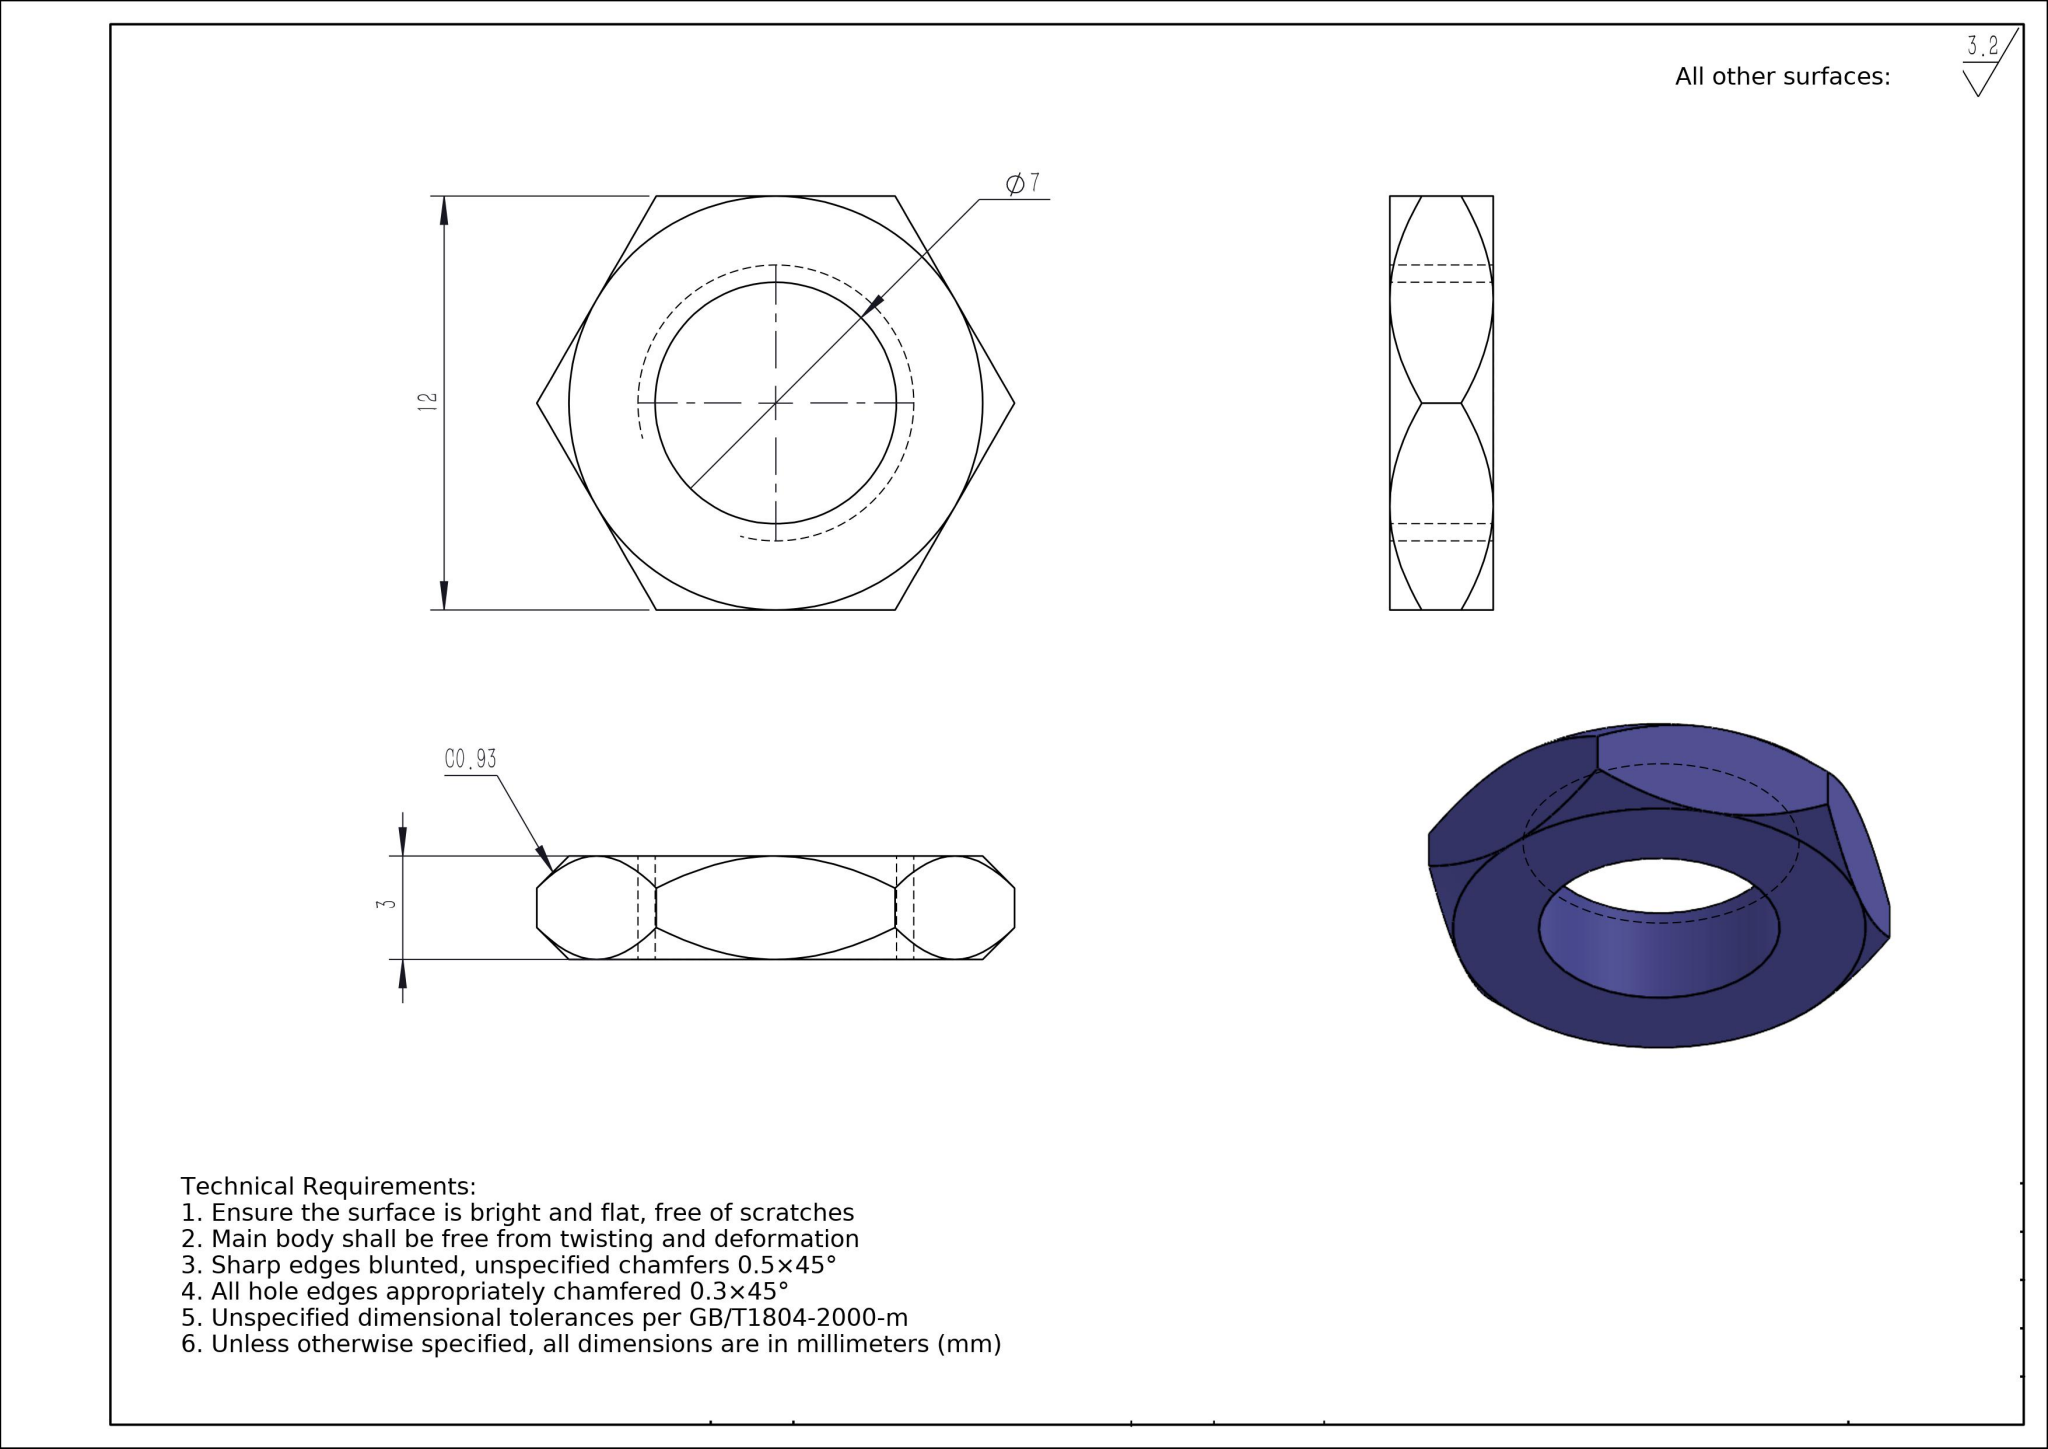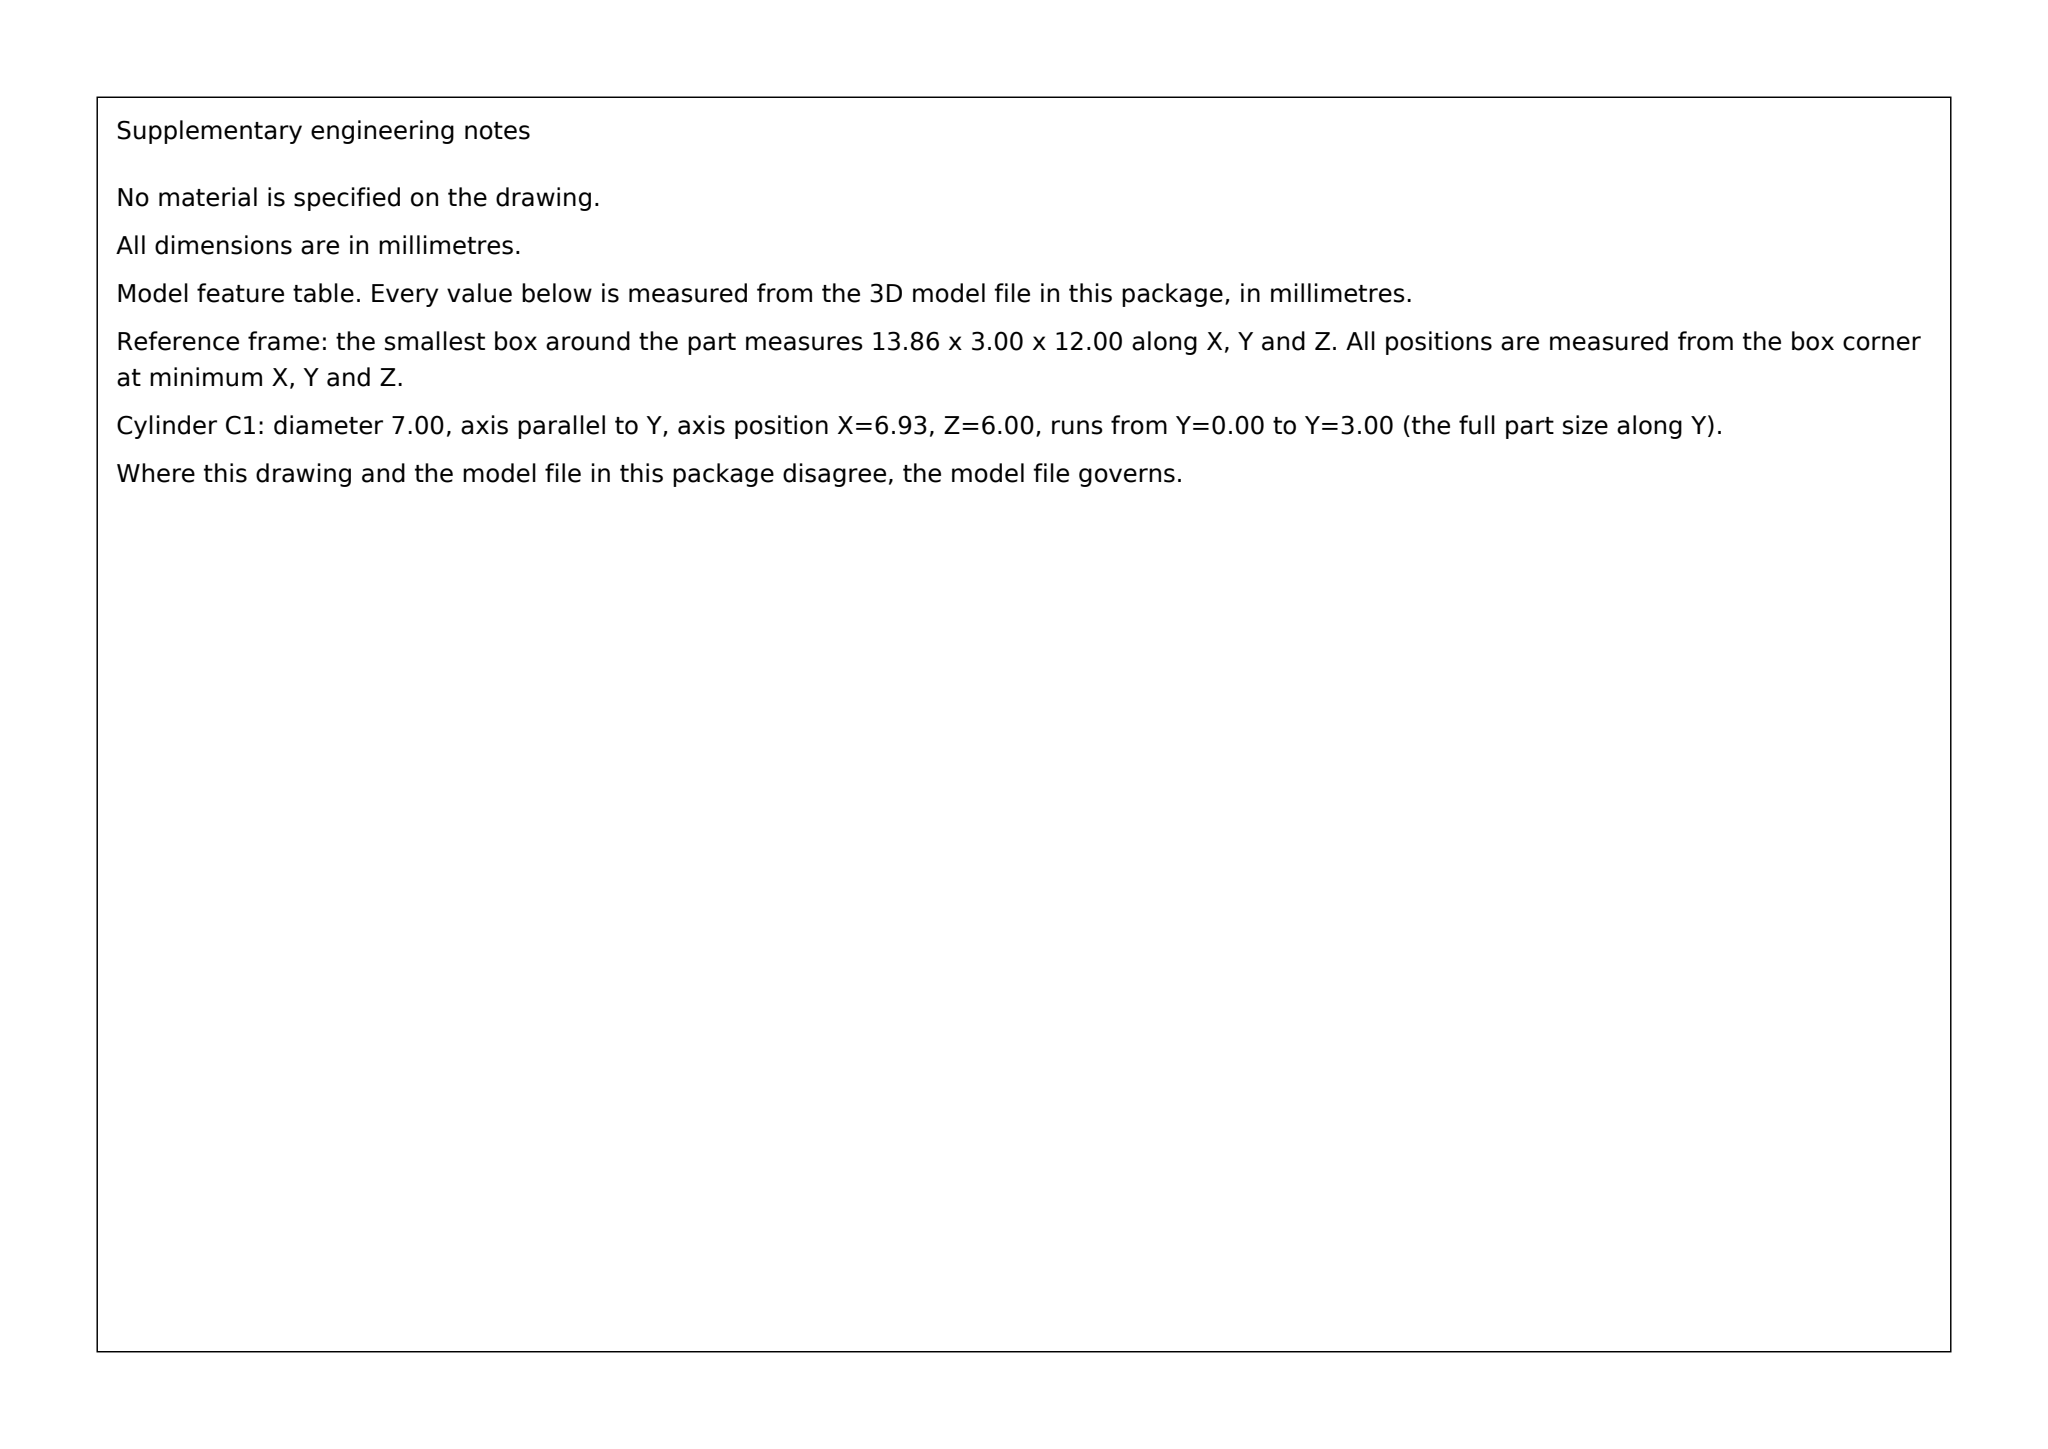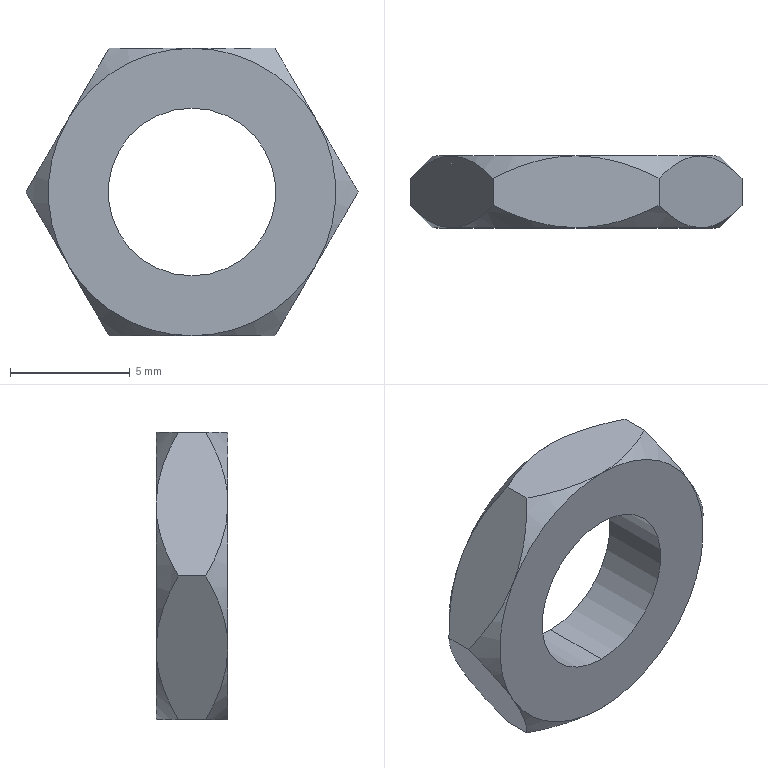Part | SolidWorks | mm | 1 solid | 22 faces | box 13.86 x 3 x 12 mm | volume 252 mm3 | cone 12 | plane 8 | cylinder 2 | commonest cylinder face diameters 7 x2
build123d program:
from build123d import *

# Parameters (mm, degrees)
BOSS_EXTRUDE2_DEPTH       = 3
M8X1_0_TAPPED_HOLE1_D     = 7
M8X1_0_TAPPED_HOLE1_DEPTH = 19
M8X1_0_TAPPED_HOLE1_TIP   = 2.103
SKETCH4_OUTSIDE_W         = 25.57
SKETCH4_OUTSIDE_H         = 23.714
SKETCH4_OUTSIDE_R         = 6
CUT_EXTRUDE1_DEPTH        = 3
CUT_EXTRUDE1_DRAFT        = -45
SKETCH5_OUTSIDE_W         = 25.57
SKETCH5_OUTSIDE_H         = 23.714
SKETCH5_OUTSIDE_R         = 6
CUT_EXTRUDE2_DEPTH        = 3
CUT_EXTRUDE2_DRAFT        = -45


with BuildPart() as part:
    # Sketch1 → Boss-Extrude2 (new body)
    with BuildSketch(Plane(origin=(0, 0, 0), x_dir=(1, 0, 0), z_dir=(0, 1, 0))):
        Polygon((6.928, 0), (3.464, 6), (-3.464, 6), (-6.928, 0), (-3.464, -6), (3.464, -6), align=None)
    extrude(amount=BOSS_EXTRUDE2_DEPTH)

    # M8x1.0 Tapped Hole1
    with Locations(Plane(origin=(0, 3, 0), x_dir=(1, 0, 0), z_dir=(0, 1, 0))):
        with Locations((0, 0)):
            Hole(M8X1_0_TAPPED_HOLE1_D / 2, depth=M8X1_0_TAPPED_HOLE1_DEPTH)
            with Locations((0, 0, -(M8X1_0_TAPPED_HOLE1_DEPTH + M8X1_0_TAPPED_HOLE1_TIP / 2))):  # 118° drill point
                Cone(0, M8X1_0_TAPPED_HOLE1_D / 2, M8X1_0_TAPPED_HOLE1_TIP, mode=Mode.SUBTRACT)


with BuildPart() as cut_extrude1_tool:
    # Sketch4 outside → Cut-Extrude1 (with draft: the straight prism first)
    with BuildSketch(Plane(origin=(0, 3, 0), x_dir=(1, 0, 0), z_dir=(0, 1, 0))):
        Rectangle(SKETCH4_OUTSIDE_W, SKETCH4_OUTSIDE_H)
        Circle(SKETCH4_OUTSIDE_R, mode=Mode.SUBTRACT)
    extrude(amount=-CUT_EXTRUDE1_DEPTH)
    # Cut-Extrude1: the draft: its side faces are tilted about the plane it starts from
    cut_extrude1_sides = [cut_extrude1_tool.faces().sort_by_distance(p)[0] for p in [
        (0, 1.5, 11.857),
        (12.785, 1.5, 0),
        (0, 1.5, -11.857),
        (-12.785, 1.5, 0),
        (-6, 1.5, 0),
    ]]
    draft(cut_extrude1_sides, Plane(origin=(0, 3, 0), x_dir=(1, 0, 0), z_dir=(0, 1, 0)), CUT_EXTRUDE1_DRAFT)


with BuildPart() as part_1:
    add(part.part)

    # Cut-Extrude1: cut by cut_extrude1_tool
    add(cut_extrude1_tool.part, mode=Mode.SUBTRACT)


with BuildPart() as cut_extrude2_tool:
    # Sketch5 outside → Cut-Extrude2 (with draft: the straight prism first)
    with BuildSketch(Plane.XZ):
        Rectangle(SKETCH5_OUTSIDE_W, SKETCH5_OUTSIDE_H)
        Circle(SKETCH5_OUTSIDE_R, mode=Mode.SUBTRACT)
    extrude(amount=-CUT_EXTRUDE2_DEPTH)
    # Cut-Extrude2: the draft: its side faces are tilted about the plane it starts from
    cut_extrude2_sides = [cut_extrude2_tool.faces().sort_by_distance(p)[0] for p in [
        (0, 1.5, -11.857),
        (12.785, 1.5, 0),
        (0, 1.5, 11.857),
        (-12.785, 1.5, 0),
        (-6, 1.5, 0),
    ]]
    draft(cut_extrude2_sides, Plane.XZ, CUT_EXTRUDE2_DRAFT)


with BuildPart() as part_2:
    add(part_1.part)

    # Cut-Extrude2: cut by cut_extrude2_tool
    add(cut_extrude2_tool.part, mode=Mode.SUBTRACT)


solid = part_2.part
STEP:
#1=CARTESIAN_POINT('',(0.,0.,-3.5));
#2=VERTEX_POINT('',#1);
#3=CARTESIAN_POINT('',(0.,0.,3.5));
#4=VERTEX_POINT('',#3);
#5=CARTESIAN_POINT('',(0.,0.,0.));
#6=DIRECTION('',(0.,1.,0.));
#7=DIRECTION('',(0.,0.,1.));
#8=AXIS2_PLACEMENT_3D('',#5,#6,#7);
#9=CIRCLE('',#8,3.5);
#10=EDGE_CURVE('',#2,#4,#9,.T.);
#11=ORIENTED_EDGE('',*,*,#10,.F.);
#12=CARTESIAN_POINT('',(0.,3.,-3.5));
#13=VERTEX_POINT('',#12);
#14=CARTESIAN_POINT('',(0.,3.,-3.5));
#15=DIRECTION('',(0.,1.,0.));
#16=VECTOR('',#15,1000.);
#17=LINE('',#14,#16);
#18=EDGE_CURVE('',#2,#13,#17,.T.);
#19=ORIENTED_EDGE('',*,*,#18,.T.);
#20=CARTESIAN_POINT('',(0.,3.,3.5));
#21=VERTEX_POINT('',#20);
#22=CARTESIAN_POINT('',(0.,3.,0.));
#23=DIRECTION('',(0.,1.,0.));
#24=DIRECTION('',(0.,0.,1.));
#25=AXIS2_PLACEMENT_3D('',#22,#23,#24);
#26=CIRCLE('',#25,3.5);
#27=EDGE_CURVE('',#13,#21,#26,.T.);
#28=ORIENTED_EDGE('',*,*,#27,.T.);
#29=CARTESIAN_POINT('',(0.,3.,3.5));
#30=DIRECTION('',(0.,1.,0.));
#31=VECTOR('',#30,1000.);
#32=LINE('',#29,#31);
#33=EDGE_CURVE('',#4,#21,#32,.T.);
#34=ORIENTED_EDGE('',*,*,#33,.F.);
#35=EDGE_LOOP('',(#11,#19,#28,#34));
#36=FACE_OUTER_BOUND('',#35,.T.);
#37=CARTESIAN_POINT('',(0.,3.,0.));
#38=DIRECTION('',(0.,1.,0.));
#39=DIRECTION('',(0.,0.,1.));
#40=AXIS2_PLACEMENT_3D('',#37,#38,#39);
#41=CYLINDRICAL_SURFACE('',#40,3.5);
#42=ADVANCED_FACE('',(#36),#41,.F.);
#43=CARTESIAN_POINT('',(6.928,0.9282,0.));
#44=VERTEX_POINT('',#43);
#45=CARTESIAN_POINT('',(5.196,0.,3.));
#46=VERTEX_POINT('',#45);
#47=CARTESIAN_POINT('',(6.928,0.9282,0.));
#48=CARTESIAN_POINT('',(6.657,0.6566,0.4704));
#49=CARTESIAN_POINT('',(6.379,0.4258,0.9515));
#50=CARTESIAN_POINT('',(5.947,0.179,1.699));
#51=CARTESIAN_POINT('',(5.801,0.1135,1.953));
#52=CARTESIAN_POINT('',(5.502,0.02381,2.471));
#53=CARTESIAN_POINT('',(5.348,0.,2.737));
#54=CARTESIAN_POINT('',(5.196,0.,3.));
#55=B_SPLINE_CURVE_WITH_KNOTS('',3,(#47,#48,#49,#50,#51,#52,#53,#54),.UNSPECIFIED.,.F.,.F.,(4,2,2,4),(0.00000025,0.001796,0.002693,0.003591),.UNSPECIFIED.);
#56=EDGE_CURVE('',#44,#46,#55,.T.);
#57=ORIENTED_EDGE('',*,*,#56,.F.);
#58=CARTESIAN_POINT('',(6.928,2.072,0.));
#59=VERTEX_POINT('',#58);
#60=CARTESIAN_POINT('',(6.928,3.,0.));
#61=DIRECTION('',(0.,-1.,0.));
#62=VECTOR('',#61,1000.);
#63=LINE('',#60,#62);
#64=EDGE_CURVE('',#59,#44,#63,.T.);
#65=ORIENTED_EDGE('',*,*,#64,.F.);
#66=CARTESIAN_POINT('',(5.196,3.,3.));
#67=VERTEX_POINT('',#66);
#68=CARTESIAN_POINT('',(5.196,3.,3.));
#69=CARTESIAN_POINT('',(5.497,3.,2.478));
#70=CARTESIAN_POINT('',(5.794,2.908,1.965));
#71=CARTESIAN_POINT('',(6.378,2.576,0.9536));
#72=CARTESIAN_POINT('',(6.657,2.343,0.4699));
#73=CARTESIAN_POINT('',(6.928,2.072,0.));
#74=B_SPLINE_CURVE_WITH_KNOTS('',3,(#68,#69,#70,#71,#72,#73),.UNSPECIFIED.,.F.,.F.,(4,2,4),(0.003591,0.005374,0.007157),.UNSPECIFIED.);
#75=EDGE_CURVE('',#67,#59,#74,.T.);
#76=ORIENTED_EDGE('',*,*,#75,.F.);
#77=CARTESIAN_POINT('',(3.464,2.072,6.));
#78=VERTEX_POINT('',#77);
#79=CARTESIAN_POINT('',(3.464,2.072,6.));
#80=CARTESIAN_POINT('',(3.736,2.343,5.53));
#81=CARTESIAN_POINT('',(4.013,2.574,5.048));
#82=CARTESIAN_POINT('',(4.445,2.821,4.301));
#83=CARTESIAN_POINT('',(4.591,2.886,4.047));
#84=CARTESIAN_POINT('',(4.89,2.976,3.529));
#85=CARTESIAN_POINT('',(5.044,3.,3.263));
#86=CARTESIAN_POINT('',(5.196,3.,3.));
#87=B_SPLINE_CURVE_WITH_KNOTS('',3,(#79,#80,#81,#82,#83,#84,#85,#86),.UNSPECIFIED.,.F.,.F.,(4,2,2,4),(0.00000025,0.001796,0.002693,0.003591),.UNSPECIFIED.);
#88=EDGE_CURVE('',#78,#67,#87,.T.);
#89=ORIENTED_EDGE('',*,*,#88,.F.);
#90=CARTESIAN_POINT('',(3.464,0.9282,6.));
#91=VERTEX_POINT('',#90);
#92=CARTESIAN_POINT('',(3.464,3.,6.));
#93=DIRECTION('',(0.,-1.,0.));
#94=VECTOR('',#93,1000.);
#95=LINE('',#92,#94);
#96=EDGE_CURVE('',#78,#91,#95,.T.);
#97=ORIENTED_EDGE('',*,*,#96,.T.);
#98=CARTESIAN_POINT('',(5.196,0.,3.));
#99=CARTESIAN_POINT('',(4.895,0.,3.522));
#100=CARTESIAN_POINT('',(4.599,0.09213,4.035));
#101=CARTESIAN_POINT('',(4.015,0.4242,5.046));
#102=CARTESIAN_POINT('',(3.735,0.6569,5.53));
#103=CARTESIAN_POINT('',(3.464,0.9282,6.));
#104=B_SPLINE_CURVE_WITH_KNOTS('',3,(#98,#99,#100,#101,#102,#103),.UNSPECIFIED.,.F.,.F.,(4,2,4),(0.003591,0.005374,0.007157),.UNSPECIFIED.);
#105=EDGE_CURVE('',#46,#91,#104,.T.);
#106=ORIENTED_EDGE('',*,*,#105,.F.);
#107=EDGE_LOOP('',(#57,#65,#76,#89,#97,#106));
#108=FACE_OUTER_BOUND('',#107,.T.);
#109=CARTESIAN_POINT('',(3.464,3.,6.));
#110=DIRECTION('',(-0.866,0.,-0.5));
#111=DIRECTION('',(-0.5,0.,0.866));
#112=AXIS2_PLACEMENT_3D('',#109,#110,#111);
#113=PLANE('',#112);
#114=ADVANCED_FACE('',(#108),#113,.F.);
#115=CARTESIAN_POINT('',(3.464,0.9282,-6.));
#116=VERTEX_POINT('',#115);
#117=CARTESIAN_POINT('',(5.196,0.,-3.));
#118=VERTEX_POINT('',#117);
#119=CARTESIAN_POINT('',(3.464,0.9282,-6.));
#120=CARTESIAN_POINT('',(3.736,0.6566,-5.53));
#121=CARTESIAN_POINT('',(4.013,0.4258,-5.048));
#122=CARTESIAN_POINT('',(4.445,0.179,-4.301));
#123=CARTESIAN_POINT('',(4.591,0.1135,-4.047));
#124=CARTESIAN_POINT('',(4.89,0.02381,-3.529));
#125=CARTESIAN_POINT('',(5.044,-0.,-3.263));
#126=CARTESIAN_POINT('',(5.196,0.,-3.));
#127=B_SPLINE_CURVE_WITH_KNOTS('',3,(#119,#120,#121,#122,#123,#124,#125,#126),.UNSPECIFIED.,.F.,.F.,(4,2,2,4),(0.00000025,0.001796,0.002693,0.003591),.UNSPECIFIED.);
#128=EDGE_CURVE('',#116,#118,#127,.T.);
#129=ORIENTED_EDGE('',*,*,#128,.F.);
#130=CARTESIAN_POINT('',(3.464,2.072,-6.));
#131=VERTEX_POINT('',#130);
#132=CARTESIAN_POINT('',(3.464,3.,-6.));
#133=DIRECTION('',(0.,-1.,0.));
#134=VECTOR('',#133,1000.);
#135=LINE('',#132,#134);
#136=EDGE_CURVE('',#131,#116,#135,.T.);
#137=ORIENTED_EDGE('',*,*,#136,.F.);
#138=CARTESIAN_POINT('',(5.196,3.,-3.));
#139=VERTEX_POINT('',#138);
#140=CARTESIAN_POINT('',(5.196,3.,-3.));
#141=CARTESIAN_POINT('',(4.895,3.,-3.522));
#142=CARTESIAN_POINT('',(4.599,2.908,-4.035));
#143=CARTESIAN_POINT('',(4.015,2.576,-5.046));
#144=CARTESIAN_POINT('',(3.735,2.343,-5.53));
#145=CARTESIAN_POINT('',(3.464,2.072,-6.));
#146=B_SPLINE_CURVE_WITH_KNOTS('',3,(#140,#141,#142,#143,#144,#145),.UNSPECIFIED.,.F.,.F.,(4,2,4),(0.003591,0.005374,0.007157),.UNSPECIFIED.);
#147=EDGE_CURVE('',#139,#131,#146,.T.);
#148=ORIENTED_EDGE('',*,*,#147,.F.);
#149=CARTESIAN_POINT('',(6.928,2.072,0.));
#150=CARTESIAN_POINT('',(6.657,2.343,-0.4704));
#151=CARTESIAN_POINT('',(6.379,2.574,-0.9515));
#152=CARTESIAN_POINT('',(5.947,2.821,-1.699));
#153=CARTESIAN_POINT('',(5.801,2.886,-1.953));
#154=CARTESIAN_POINT('',(5.502,2.976,-2.471));
#155=CARTESIAN_POINT('',(5.348,3.,-2.737));
#156=CARTESIAN_POINT('',(5.196,3.,-3.));
#157=B_SPLINE_CURVE_WITH_KNOTS('',3,(#149,#150,#151,#152,#153,#154,#155,#156),.UNSPECIFIED.,.F.,.F.,(4,2,2,4),(0.00000025,0.001796,0.002693,0.003591),.UNSPECIFIED.);
#158=EDGE_CURVE('',#59,#139,#157,.T.);
#159=ORIENTED_EDGE('',*,*,#158,.F.);
#160=ORIENTED_EDGE('',*,*,#64,.T.);
#161=CARTESIAN_POINT('',(5.196,0.,-3.));
#162=CARTESIAN_POINT('',(5.497,-0.,-2.478));
#163=CARTESIAN_POINT('',(5.794,0.09213,-1.965));
#164=CARTESIAN_POINT('',(6.378,0.4242,-0.9536));
#165=CARTESIAN_POINT('',(6.657,0.6569,-0.4699));
#166=CARTESIAN_POINT('',(6.928,0.9282,0.));
#167=B_SPLINE_CURVE_WITH_KNOTS('',3,(#161,#162,#163,#164,#165,#166),.UNSPECIFIED.,.F.,.F.,(4,2,4),(0.003591,0.005374,0.007157),.UNSPECIFIED.);
#168=EDGE_CURVE('',#118,#44,#167,.T.);
#169=ORIENTED_EDGE('',*,*,#168,.F.);
#170=EDGE_LOOP('',(#129,#137,#148,#159,#160,#169));
#171=FACE_OUTER_BOUND('',#170,.T.);
#172=CARTESIAN_POINT('',(6.928,3.,0.));
#173=DIRECTION('',(-0.866,0.,0.5));
#174=DIRECTION('',(0.5,0.,0.866));
#175=AXIS2_PLACEMENT_3D('',#172,#173,#174);
#176=PLANE('',#175);
#177=ADVANCED_FACE('',(#171),#176,.F.);
#178=CARTESIAN_POINT('',(-3.464,0.9282,-6.));
#179=VERTEX_POINT('',#178);
#180=CARTESIAN_POINT('',(0.,0.,-6.));
#181=VERTEX_POINT('',#180);
#182=CARTESIAN_POINT('',(-3.464,0.9282,-6.));
#183=CARTESIAN_POINT('',(-2.927,0.6597,-6.));
#184=CARTESIAN_POINT('',(-2.362,0.4243,-6.));
#185=CARTESIAN_POINT('',(-1.496,0.1774,-6.));
#186=CARTESIAN_POINT('',(-1.203,0.1123,-6.));
#187=CARTESIAN_POINT('',(-0.6083,0.02359,-6.));
#188=CARTESIAN_POINT('',(-0.3039,-0.,-6.));
#189=CARTESIAN_POINT('',(0.,0.,-6.));
#190=B_SPLINE_CURVE_WITH_KNOTS('',3,(#182,#183,#184,#185,#186,#187,#188,#189),.UNSPECIFIED.,.F.,.F.,(4,2,2,4),(0.006042,0.00783,0.008725,0.009619),.UNSPECIFIED.);
#191=EDGE_CURVE('',#179,#181,#190,.T.);
#192=ORIENTED_EDGE('',*,*,#191,.F.);
#193=CARTESIAN_POINT('',(-3.464,2.072,-6.));
#194=VERTEX_POINT('',#193);
#195=CARTESIAN_POINT('',(-3.464,3.,-6.));
#196=DIRECTION('',(0.,-1.,0.));
#197=VECTOR('',#196,1000.);
#198=LINE('',#195,#197);
#199=EDGE_CURVE('',#194,#179,#198,.T.);
#200=ORIENTED_EDGE('',*,*,#199,.F.);
#201=CARTESIAN_POINT('',(0.,3.,-6.));
#202=VERTEX_POINT('',#201);
#203=CARTESIAN_POINT('',(0.,3.,-6.));
#204=CARTESIAN_POINT('',(-0.3039,3.,-6.));
#205=CARTESIAN_POINT('',(-0.6083,2.976,-6.));
#206=CARTESIAN_POINT('',(-1.203,2.888,-6.));
#207=CARTESIAN_POINT('',(-1.496,2.823,-6.));
#208=CARTESIAN_POINT('',(-2.362,2.576,-6.));
#209=CARTESIAN_POINT('',(-2.927,2.34,-6.));
#210=CARTESIAN_POINT('',(-3.464,2.072,-6.));
#211=B_SPLINE_CURVE_WITH_KNOTS('',3,(#203,#204,#205,#206,#207,#208,#209,#210),.UNSPECIFIED.,.F.,.F.,(4,2,2,4),(0.007239,0.008136,0.009033,0.01083),.UNSPECIFIED.);
#212=EDGE_CURVE('',#202,#194,#211,.T.);
#213=ORIENTED_EDGE('',*,*,#212,.F.);
#214=CARTESIAN_POINT('',(3.464,2.072,-6.));
#215=CARTESIAN_POINT('',(3.196,2.206,-6.));
#216=CARTESIAN_POINT('',(2.923,2.331,-6.));
#217=CARTESIAN_POINT('',(2.362,2.557,-6.));
#218=CARTESIAN_POINT('',(2.073,2.658,-6.));
#219=CARTESIAN_POINT('',(1.202,2.906,-6.));
#220=CARTESIAN_POINT('',(0.6086,3.,-6.));
#221=CARTESIAN_POINT('',(0.,3.,-6.));
#222=B_SPLINE_CURVE_WITH_KNOTS('',3,(#214,#215,#216,#217,#218,#219,#220,#221),.UNSPECIFIED.,.F.,.F.,(4,2,2,4),(0.003647,0.004545,0.005443,0.007239),.UNSPECIFIED.);
#223=EDGE_CURVE('',#131,#202,#222,.T.);
#224=ORIENTED_EDGE('',*,*,#223,.F.);
#225=ORIENTED_EDGE('',*,*,#136,.T.);
#226=CARTESIAN_POINT('',(0.,0.,-6.));
#227=CARTESIAN_POINT('',(0.6086,-0.,-6.));
#228=CARTESIAN_POINT('',(1.202,0.09373,-6.));
#229=CARTESIAN_POINT('',(2.073,0.3419,-6.));
#230=CARTESIAN_POINT('',(2.362,0.443,-6.));
#231=CARTESIAN_POINT('',(2.923,0.669,-6.));
#232=CARTESIAN_POINT('',(3.196,0.7941,-6.));
#233=CARTESIAN_POINT('',(3.464,0.9282,-6.));
#234=B_SPLINE_CURVE_WITH_KNOTS('',3,(#226,#227,#228,#229,#230,#231,#232,#233),.UNSPECIFIED.,.F.,.F.,(4,2,2,4),(0.009619,0.01141,0.0123,0.0132),.UNSPECIFIED.);
#235=EDGE_CURVE('',#181,#116,#234,.T.);
#236=ORIENTED_EDGE('',*,*,#235,.F.);
#237=EDGE_LOOP('',(#192,#200,#213,#224,#225,#236));
#238=FACE_OUTER_BOUND('',#237,.T.);
#239=CARTESIAN_POINT('',(3.464,3.,-6.));
#240=DIRECTION('',(0.,0.,1.));
#241=DIRECTION('',(1.,0.,0.));
#242=AXIS2_PLACEMENT_3D('',#239,#240,#241);
#243=PLANE('',#242);
#244=ADVANCED_FACE('',(#238),#243,.F.);
#245=CARTESIAN_POINT('',(-6.928,0.9282,0.));
#246=VERTEX_POINT('',#245);
#247=CARTESIAN_POINT('',(-5.196,0.,-3.));
#248=VERTEX_POINT('',#247);
#249=CARTESIAN_POINT('',(-6.928,0.9282,0.));
#250=CARTESIAN_POINT('',(-6.657,0.6566,-0.4704));
#251=CARTESIAN_POINT('',(-6.379,0.4258,-0.9515));
#252=CARTESIAN_POINT('',(-5.947,0.179,-1.699));
#253=CARTESIAN_POINT('',(-5.801,0.1135,-1.953));
#254=CARTESIAN_POINT('',(-5.502,0.02381,-2.471));
#255=CARTESIAN_POINT('',(-5.348,0.,-2.737));
#256=CARTESIAN_POINT('',(-5.196,0.,-3.));
#257=B_SPLINE_CURVE_WITH_KNOTS('',3,(#249,#250,#251,#252,#253,#254,#255,#256),.UNSPECIFIED.,.F.,.F.,(4,2,2,4),(0.00000025,0.001796,0.002693,0.003591),.UNSPECIFIED.);
#258=EDGE_CURVE('',#246,#248,#257,.T.);
#259=ORIENTED_EDGE('',*,*,#258,.F.);
#260=CARTESIAN_POINT('',(-6.928,2.072,0.));
#261=VERTEX_POINT('',#260);
#262=CARTESIAN_POINT('',(-6.928,3.,-0.));
#263=DIRECTION('',(0.,-1.,0.));
#264=VECTOR('',#263,1000.);
#265=LINE('',#262,#264);
#266=EDGE_CURVE('',#261,#246,#265,.T.);
#267=ORIENTED_EDGE('',*,*,#266,.F.);
#268=CARTESIAN_POINT('',(-5.196,3.,-3.));
#269=VERTEX_POINT('',#268);
#270=CARTESIAN_POINT('',(-5.196,3.,-3.));
#271=CARTESIAN_POINT('',(-5.497,3.,-2.478));
#272=CARTESIAN_POINT('',(-5.794,2.908,-1.965));
#273=CARTESIAN_POINT('',(-6.378,2.576,-0.9536));
#274=CARTESIAN_POINT('',(-6.657,2.343,-0.4699));
#275=CARTESIAN_POINT('',(-6.928,2.072,0.));
#276=B_SPLINE_CURVE_WITH_KNOTS('',3,(#270,#271,#272,#273,#274,#275),.UNSPECIFIED.,.F.,.F.,(4,2,4),(0.003591,0.005374,0.007157),.UNSPECIFIED.);
#277=EDGE_CURVE('',#269,#261,#276,.T.);
#278=ORIENTED_EDGE('',*,*,#277,.F.);
#279=CARTESIAN_POINT('',(-3.464,2.072,-6.));
#280=CARTESIAN_POINT('',(-3.736,2.343,-5.53));
#281=CARTESIAN_POINT('',(-4.013,2.574,-5.048));
#282=CARTESIAN_POINT('',(-4.445,2.821,-4.301));
#283=CARTESIAN_POINT('',(-4.591,2.886,-4.047));
#284=CARTESIAN_POINT('',(-4.89,2.976,-3.529));
#285=CARTESIAN_POINT('',(-5.044,3.,-3.263));
#286=CARTESIAN_POINT('',(-5.196,3.,-3.));
#287=B_SPLINE_CURVE_WITH_KNOTS('',3,(#279,#280,#281,#282,#283,#284,#285,#286),.UNSPECIFIED.,.F.,.F.,(4,2,2,4),(0.00000025,0.001796,0.002693,0.003591),.UNSPECIFIED.);
#288=EDGE_CURVE('',#194,#269,#287,.T.);
#289=ORIENTED_EDGE('',*,*,#288,.F.);
#290=ORIENTED_EDGE('',*,*,#199,.T.);
#291=CARTESIAN_POINT('',(-5.196,0.,-3.));
#292=CARTESIAN_POINT('',(-4.895,0.,-3.522));
#293=CARTESIAN_POINT('',(-4.599,0.09213,-4.035));
#294=CARTESIAN_POINT('',(-4.015,0.4242,-5.046));
#295=CARTESIAN_POINT('',(-3.735,0.6569,-5.53));
#296=CARTESIAN_POINT('',(-3.464,0.9282,-6.));
#297=B_SPLINE_CURVE_WITH_KNOTS('',3,(#291,#292,#293,#294,#295,#296),.UNSPECIFIED.,.F.,.F.,(4,2,4),(0.003591,0.005374,0.007157),.UNSPECIFIED.);
#298=EDGE_CURVE('',#248,#179,#297,.T.);
#299=ORIENTED_EDGE('',*,*,#298,.F.);
#300=EDGE_LOOP('',(#259,#267,#278,#289,#290,#299));
#301=FACE_OUTER_BOUND('',#300,.T.);
#302=CARTESIAN_POINT('',(-3.464,3.,-6.));
#303=DIRECTION('',(0.866,0.,0.5));
#304=DIRECTION('',(0.5,0.,-0.866));
#305=AXIS2_PLACEMENT_3D('',#302,#303,#304);
#306=PLANE('',#305);
#307=ADVANCED_FACE('',(#301),#306,.F.);
#308=CARTESIAN_POINT('',(-3.464,0.9282,6.));
#309=VERTEX_POINT('',#308);
#310=CARTESIAN_POINT('',(-5.196,0.,3.));
#311=VERTEX_POINT('',#310);
#312=CARTESIAN_POINT('',(-3.464,0.9282,6.));
#313=CARTESIAN_POINT('',(-3.736,0.6566,5.53));
#314=CARTESIAN_POINT('',(-4.013,0.4258,5.048));
#315=CARTESIAN_POINT('',(-4.445,0.179,4.301));
#316=CARTESIAN_POINT('',(-4.591,0.1135,4.047));
#317=CARTESIAN_POINT('',(-4.89,0.02381,3.529));
#318=CARTESIAN_POINT('',(-5.044,0.,3.263));
#319=CARTESIAN_POINT('',(-5.196,0.,3.));
#320=B_SPLINE_CURVE_WITH_KNOTS('',3,(#312,#313,#314,#315,#316,#317,#318,#319),.UNSPECIFIED.,.F.,.F.,(4,2,2,4),(0.00000025,0.001796,0.002693,0.003591),.UNSPECIFIED.);
#321=EDGE_CURVE('',#309,#311,#320,.T.);
#322=ORIENTED_EDGE('',*,*,#321,.F.);
#323=CARTESIAN_POINT('',(-3.464,2.072,6.));
#324=VERTEX_POINT('',#323);
#325=CARTESIAN_POINT('',(-3.464,3.,6.));
#326=DIRECTION('',(0.,-1.,0.));
#327=VECTOR('',#326,1000.);
#328=LINE('',#325,#327);
#329=EDGE_CURVE('',#324,#309,#328,.T.);
#330=ORIENTED_EDGE('',*,*,#329,.F.);
#331=CARTESIAN_POINT('',(-5.196,3.,3.));
#332=VERTEX_POINT('',#331);
#333=CARTESIAN_POINT('',(-5.196,3.,3.));
#334=CARTESIAN_POINT('',(-4.895,3.,3.522));
#335=CARTESIAN_POINT('',(-4.599,2.908,4.035));
#336=CARTESIAN_POINT('',(-4.015,2.576,5.046));
#337=CARTESIAN_POINT('',(-3.735,2.343,5.53));
#338=CARTESIAN_POINT('',(-3.464,2.072,6.));
#339=B_SPLINE_CURVE_WITH_KNOTS('',3,(#333,#334,#335,#336,#337,#338),.UNSPECIFIED.,.F.,.F.,(4,2,4),(0.003591,0.005374,0.007157),.UNSPECIFIED.);
#340=EDGE_CURVE('',#332,#324,#339,.T.);
#341=ORIENTED_EDGE('',*,*,#340,.F.);
#342=CARTESIAN_POINT('',(-6.928,2.072,0.));
#343=CARTESIAN_POINT('',(-6.657,2.343,0.4704));
#344=CARTESIAN_POINT('',(-6.379,2.574,0.9515));
#345=CARTESIAN_POINT('',(-5.947,2.821,1.699));
#346=CARTESIAN_POINT('',(-5.801,2.886,1.953));
#347=CARTESIAN_POINT('',(-5.502,2.976,2.471));
#348=CARTESIAN_POINT('',(-5.348,3.,2.737));
#349=CARTESIAN_POINT('',(-5.196,3.,3.));
#350=B_SPLINE_CURVE_WITH_KNOTS('',3,(#342,#343,#344,#345,#346,#347,#348,#349),.UNSPECIFIED.,.F.,.F.,(4,2,2,4),(0.00000025,0.001796,0.002693,0.003591),.UNSPECIFIED.);
#351=EDGE_CURVE('',#261,#332,#350,.T.);
#352=ORIENTED_EDGE('',*,*,#351,.F.);
#353=ORIENTED_EDGE('',*,*,#266,.T.);
#354=CARTESIAN_POINT('',(-5.196,0.,3.));
#355=CARTESIAN_POINT('',(-5.497,0.,2.478));
#356=CARTESIAN_POINT('',(-5.794,0.09213,1.965));
#357=CARTESIAN_POINT('',(-6.378,0.4242,0.9536));
#358=CARTESIAN_POINT('',(-6.657,0.6569,0.4699));
#359=CARTESIAN_POINT('',(-6.928,0.9282,0.));
#360=B_SPLINE_CURVE_WITH_KNOTS('',3,(#354,#355,#356,#357,#358,#359),.UNSPECIFIED.,.F.,.F.,(4,2,4),(0.003591,0.005374,0.007157),.UNSPECIFIED.);
#361=EDGE_CURVE('',#311,#246,#360,.T.);
#362=ORIENTED_EDGE('',*,*,#361,.F.);
#363=EDGE_LOOP('',(#322,#330,#341,#352,#353,#362));
#364=FACE_OUTER_BOUND('',#363,.T.);
#365=CARTESIAN_POINT('',(-6.928,3.,-0.));
#366=DIRECTION('',(0.866,0.,-0.5));
#367=DIRECTION('',(-0.5,0.,-0.866));
#368=AXIS2_PLACEMENT_3D('',#365,#366,#367);
#369=PLANE('',#368);
#370=ADVANCED_FACE('',(#364),#369,.F.);
#371=CARTESIAN_POINT('',(-0.,0.,6.));
#372=VERTEX_POINT('',#371);
#373=CARTESIAN_POINT('',(3.464,0.9282,6.));
#374=CARTESIAN_POINT('',(3.196,0.7941,6.));
#375=CARTESIAN_POINT('',(2.923,0.669,6.));
#376=CARTESIAN_POINT('',(2.362,0.443,6.));
#377=CARTESIAN_POINT('',(2.073,0.3419,6.));
#378=CARTESIAN_POINT('',(1.202,0.09373,6.));
#379=CARTESIAN_POINT('',(0.6086,-0.,6.));
#380=CARTESIAN_POINT('',(-0.,0.,6.));
#381=B_SPLINE_CURVE_WITH_KNOTS('',3,(#373,#374,#375,#376,#377,#378,#379,#380),.UNSPECIFIED.,.F.,.F.,(4,2,2,4),(0.003647,0.004545,0.005443,0.007239),.UNSPECIFIED.);
#382=EDGE_CURVE('',#91,#372,#381,.T.);
#383=ORIENTED_EDGE('',*,*,#382,.F.);
#384=ORIENTED_EDGE('',*,*,#96,.F.);
#385=CARTESIAN_POINT('',(-0.,3.,6.));
#386=VERTEX_POINT('',#385);
#387=CARTESIAN_POINT('',(-0.,3.,6.));
#388=CARTESIAN_POINT('',(0.6086,3.,6.));
#389=CARTESIAN_POINT('',(1.202,2.906,6.));
#390=CARTESIAN_POINT('',(2.073,2.658,6.));
#391=CARTESIAN_POINT('',(2.362,2.557,6.));
#392=CARTESIAN_POINT('',(2.923,2.331,6.));
#393=CARTESIAN_POINT('',(3.196,2.206,6.));
#394=CARTESIAN_POINT('',(3.464,2.072,6.));
#395=B_SPLINE_CURVE_WITH_KNOTS('',3,(#387,#388,#389,#390,#391,#392,#393,#394),.UNSPECIFIED.,.F.,.F.,(4,2,2,4),(0.009619,0.01141,0.0123,0.0132),.UNSPECIFIED.);
#396=EDGE_CURVE('',#386,#78,#395,.T.);
#397=ORIENTED_EDGE('',*,*,#396,.F.);
#398=CARTESIAN_POINT('',(-3.464,2.072,6.));
#399=CARTESIAN_POINT('',(-2.927,2.34,6.));
#400=CARTESIAN_POINT('',(-2.362,2.576,6.));
#401=CARTESIAN_POINT('',(-1.496,2.823,6.));
#402=CARTESIAN_POINT('',(-1.203,2.888,6.));
#403=CARTESIAN_POINT('',(-0.6083,2.976,6.));
#404=CARTESIAN_POINT('',(-0.3039,3.,6.));
#405=CARTESIAN_POINT('',(-0.,3.,6.));
#406=B_SPLINE_CURVE_WITH_KNOTS('',3,(#398,#399,#400,#401,#402,#403,#404,#405),.UNSPECIFIED.,.F.,.F.,(4,2,2,4),(0.006042,0.00783,0.008725,0.009619),.UNSPECIFIED.);
#407=EDGE_CURVE('',#324,#386,#406,.T.);
#408=ORIENTED_EDGE('',*,*,#407,.F.);
#409=ORIENTED_EDGE('',*,*,#329,.T.);
#410=CARTESIAN_POINT('',(-0.,0.,6.));
#411=CARTESIAN_POINT('',(-0.3039,-0.,6.));
#412=CARTESIAN_POINT('',(-0.6083,0.02359,6.));
#413=CARTESIAN_POINT('',(-1.203,0.1123,6.));
#414=CARTESIAN_POINT('',(-1.496,0.1774,6.));
#415=CARTESIAN_POINT('',(-2.362,0.4243,6.));
#416=CARTESIAN_POINT('',(-2.927,0.6597,6.));
#417=CARTESIAN_POINT('',(-3.464,0.9282,6.));
#418=B_SPLINE_CURVE_WITH_KNOTS('',3,(#410,#411,#412,#413,#414,#415,#416,#417),.UNSPECIFIED.,.F.,.F.,(4,2,2,4),(0.007239,0.008136,0.009033,0.01083),.UNSPECIFIED.);
#419=EDGE_CURVE('',#372,#309,#418,.T.);
#420=ORIENTED_EDGE('',*,*,#419,.F.);
#421=EDGE_LOOP('',(#383,#384,#397,#408,#409,#420));
#422=FACE_OUTER_BOUND('',#421,.T.);
#423=CARTESIAN_POINT('',(-3.464,3.,6.));
#424=DIRECTION('',(0.,0.,-1.));
#425=DIRECTION('',(-1.,0.,-0.));
#426=AXIS2_PLACEMENT_3D('',#423,#424,#425);
#427=PLANE('',#426);
#428=ADVANCED_FACE('',(#422),#427,.F.);
#429=CARTESIAN_POINT('',(0.,0.,0.));
#430=DIRECTION('',(0.,1.,0.));
#431=DIRECTION('',(0.,0.,1.));
#432=AXIS2_PLACEMENT_3D('',#429,#430,#431);
#433=CIRCLE('',#432,3.5);
#434=EDGE_CURVE('',#4,#2,#433,.T.);
#435=ORIENTED_EDGE('',*,*,#434,.T.);
#436=ORIENTED_EDGE('',*,*,#10,.T.);
#437=EDGE_LOOP('',(#435,#436));
#438=FACE_BOUND('',#437,.T.);
#439=CARTESIAN_POINT('',(0.,0.,0.));
#440=DIRECTION('',(0.,1.,0.));
#441=DIRECTION('',(0.,0.,1.));
#442=AXIS2_PLACEMENT_3D('',#439,#440,#441);
#443=CIRCLE('',#442,6.);
#444=EDGE_CURVE('',#372,#46,#443,.T.);
#445=ORIENTED_EDGE('',*,*,#444,.F.);
#446=CARTESIAN_POINT('',(0.,0.,0.));
#447=DIRECTION('',(0.,1.,0.));
#448=DIRECTION('',(0.,0.,1.));
#449=AXIS2_PLACEMENT_3D('',#446,#447,#448);
#450=CIRCLE('',#449,6.);
#451=EDGE_CURVE('',#311,#372,#450,.T.);
#452=ORIENTED_EDGE('',*,*,#451,.F.);
#453=CARTESIAN_POINT('',(0.,0.,0.));
#454=DIRECTION('',(0.,1.,0.));
#455=DIRECTION('',(0.,0.,1.));
#456=AXIS2_PLACEMENT_3D('',#453,#454,#455);
#457=CIRCLE('',#456,6.);
#458=EDGE_CURVE('',#248,#311,#457,.T.);
#459=ORIENTED_EDGE('',*,*,#458,.F.);
#460=CARTESIAN_POINT('',(0.,0.,0.));
#461=DIRECTION('',(0.,1.,0.));
#462=DIRECTION('',(0.,0.,1.));
#463=AXIS2_PLACEMENT_3D('',#460,#461,#462);
#464=CIRCLE('',#463,6.);
#465=EDGE_CURVE('',#181,#248,#464,.T.);
#466=ORIENTED_EDGE('',*,*,#465,.F.);
#467=CARTESIAN_POINT('',(0.,0.,0.));
#468=DIRECTION('',(0.,-1.,0.));
#469=DIRECTION('',(0.,0.,-1.));
#470=AXIS2_PLACEMENT_3D('',#467,#468,#469);
#471=CIRCLE('',#470,6.);
#472=EDGE_CURVE('',#181,#118,#471,.T.);
#473=ORIENTED_EDGE('',*,*,#472,.T.);
#474=CARTESIAN_POINT('',(0.,0.,0.));
#475=DIRECTION('',(0.,1.,0.));
#476=DIRECTION('',(0.,0.,1.));
#477=AXIS2_PLACEMENT_3D('',#474,#475,#476);
#478=CIRCLE('',#477,6.);
#479=EDGE_CURVE('',#46,#118,#478,.T.);
#480=ORIENTED_EDGE('',*,*,#479,.F.);
#481=EDGE_LOOP('',(#445,#452,#459,#466,#473,#480));
#482=FACE_OUTER_BOUND('',#481,.T.);
#483=CARTESIAN_POINT('',(0.,0.,0.));
#484=DIRECTION('',(0.,1.,0.));
#485=DIRECTION('',(0.,0.,1.));
#486=AXIS2_PLACEMENT_3D('',#483,#484,#485);
#487=PLANE('',#486);
#488=ADVANCED_FACE('',(#438,#482),#487,.F.);
#489=CARTESIAN_POINT('',(0.,3.,0.));
#490=DIRECTION('',(0.,1.,0.));
#491=DIRECTION('',(0.,0.,1.));
#492=AXIS2_PLACEMENT_3D('',#489,#490,#491);
#493=CIRCLE('',#492,3.5);
#494=EDGE_CURVE('',#21,#13,#493,.T.);
#495=ORIENTED_EDGE('',*,*,#494,.F.);
#496=ORIENTED_EDGE('',*,*,#27,.F.);
#497=EDGE_LOOP('',(#495,#496));
#498=FACE_BOUND('',#497,.T.);
#499=CARTESIAN_POINT('',(0.,3.,0.));
#500=DIRECTION('',(0.,1.,0.));
#501=DIRECTION('',(0.,0.,1.));
#502=AXIS2_PLACEMENT_3D('',#499,#500,#501);
#503=CIRCLE('',#502,6.);
#504=EDGE_CURVE('',#332,#386,#503,.T.);
#505=ORIENTED_EDGE('',*,*,#504,.T.);
#506=CARTESIAN_POINT('',(0.,3.,0.));
#507=DIRECTION('',(0.,1.,0.));
#508=DIRECTION('',(0.,0.,1.));
#509=AXIS2_PLACEMENT_3D('',#506,#507,#508);
#510=CIRCLE('',#509,6.);
#511=EDGE_CURVE('',#386,#67,#510,.T.);
#512=ORIENTED_EDGE('',*,*,#511,.T.);
#513=CARTESIAN_POINT('',(0.,3.,0.));
#514=DIRECTION('',(0.,1.,0.));
#515=DIRECTION('',(0.,0.,1.));
#516=AXIS2_PLACEMENT_3D('',#513,#514,#515);
#517=CIRCLE('',#516,6.);
#518=EDGE_CURVE('',#67,#139,#517,.T.);
#519=ORIENTED_EDGE('',*,*,#518,.T.);
#520=CARTESIAN_POINT('',(0.,3.,0.));
#521=DIRECTION('',(0.,1.,0.));
#522=DIRECTION('',(0.,0.,1.));
#523=AXIS2_PLACEMENT_3D('',#520,#521,#522);
#524=CIRCLE('',#523,6.);
#525=EDGE_CURVE('',#139,#202,#524,.T.);
#526=ORIENTED_EDGE('',*,*,#525,.T.);
#527=CARTESIAN_POINT('',(0.,3.,0.));
#528=DIRECTION('',(0.,1.,0.));
#529=DIRECTION('',(0.,0.,1.));
#530=AXIS2_PLACEMENT_3D('',#527,#528,#529);
#531=CIRCLE('',#530,6.);
#532=EDGE_CURVE('',#202,#269,#531,.T.);
#533=ORIENTED_EDGE('',*,*,#532,.T.);
#534=CARTESIAN_POINT('',(0.,3.,0.));
#535=DIRECTION('',(0.,1.,0.));
#536=DIRECTION('',(0.,0.,1.));
#537=AXIS2_PLACEMENT_3D('',#534,#535,#536);
#538=CIRCLE('',#537,6.);
#539=EDGE_CURVE('',#269,#332,#538,.T.);
#540=ORIENTED_EDGE('',*,*,#539,.T.);
#541=EDGE_LOOP('',(#505,#512,#519,#526,#533,#540));
#542=FACE_OUTER_BOUND('',#541,.T.);
#543=CARTESIAN_POINT('',(0.,3.,0.));
#544=DIRECTION('',(0.,1.,0.));
#545=DIRECTION('',(0.,0.,1.));
#546=AXIS2_PLACEMENT_3D('',#543,#544,#545);
#547=PLANE('',#546);
#548=ADVANCED_FACE('',(#498,#542),#547,.T.);
#549=ORIENTED_EDGE('',*,*,#18,.F.);
#550=ORIENTED_EDGE('',*,*,#434,.F.);
#551=ORIENTED_EDGE('',*,*,#33,.T.);
#552=ORIENTED_EDGE('',*,*,#494,.T.);
#553=EDGE_LOOP('',(#549,#550,#551,#552));
#554=FACE_OUTER_BOUND('',#553,.T.);
#555=CARTESIAN_POINT('',(0.,3.,0.));
#556=DIRECTION('',(0.,1.,0.));
#557=DIRECTION('',(0.,0.,1.));
#558=AXIS2_PLACEMENT_3D('',#555,#556,#557);
#559=CYLINDRICAL_SURFACE('',#558,3.5);
#560=ADVANCED_FACE('',(#554),#559,.F.);
#561=ORIENTED_EDGE('',*,*,#340,.T.);
#562=ORIENTED_EDGE('',*,*,#407,.T.);
#563=ORIENTED_EDGE('',*,*,#504,.F.);
#564=EDGE_LOOP('',(#561,#562,#563));
#565=FACE_OUTER_BOUND('',#564,.T.);
#566=CARTESIAN_POINT('',(0.,3.,0.));
#567=DIRECTION('',(0.,-1.,0.));
#568=DIRECTION('',(0.,0.,1.));
#569=AXIS2_PLACEMENT_3D('',#566,#567,#568);
#570=CONICAL_SURFACE('',#569,6.,0.7854);
#571=ADVANCED_FACE('',(#565),#570,.T.);
#572=ORIENTED_EDGE('',*,*,#277,.T.);
#573=ORIENTED_EDGE('',*,*,#351,.T.);
#574=ORIENTED_EDGE('',*,*,#539,.F.);
#575=EDGE_LOOP('',(#572,#573,#574));
#576=FACE_OUTER_BOUND('',#575,.T.);
#577=CARTESIAN_POINT('',(0.,3.,0.));
#578=DIRECTION('',(0.,-1.,0.));
#579=DIRECTION('',(0.,0.,1.));
#580=AXIS2_PLACEMENT_3D('',#577,#578,#579);
#581=CONICAL_SURFACE('',#580,6.,0.7854);
#582=ADVANCED_FACE('',(#576),#581,.T.);
#583=ORIENTED_EDGE('',*,*,#212,.T.);
#584=ORIENTED_EDGE('',*,*,#288,.T.);
#585=ORIENTED_EDGE('',*,*,#532,.F.);
#586=EDGE_LOOP('',(#583,#584,#585));
#587=FACE_OUTER_BOUND('',#586,.T.);
#588=CARTESIAN_POINT('',(0.,3.,0.));
#589=DIRECTION('',(0.,-1.,0.));
#590=DIRECTION('',(0.,0.,1.));
#591=AXIS2_PLACEMENT_3D('',#588,#589,#590);
#592=CONICAL_SURFACE('',#591,6.,0.7854);
#593=ADVANCED_FACE('',(#587),#592,.T.);
#594=ORIENTED_EDGE('',*,*,#147,.T.);
#595=ORIENTED_EDGE('',*,*,#223,.T.);
#596=ORIENTED_EDGE('',*,*,#525,.F.);
#597=EDGE_LOOP('',(#594,#595,#596));
#598=FACE_OUTER_BOUND('',#597,.T.);
#599=CARTESIAN_POINT('',(0.,3.,0.));
#600=DIRECTION('',(0.,-1.,0.));
#601=DIRECTION('',(0.,0.,1.));
#602=AXIS2_PLACEMENT_3D('',#599,#600,#601);
#603=CONICAL_SURFACE('',#602,6.,0.7854);
#604=ADVANCED_FACE('',(#598),#603,.T.);
#605=ORIENTED_EDGE('',*,*,#75,.T.);
#606=ORIENTED_EDGE('',*,*,#158,.T.);
#607=ORIENTED_EDGE('',*,*,#518,.F.);
#608=EDGE_LOOP('',(#605,#606,#607));
#609=FACE_OUTER_BOUND('',#608,.T.);
#610=CARTESIAN_POINT('',(0.,3.,0.));
#611=DIRECTION('',(0.,-1.,0.));
#612=DIRECTION('',(0.,0.,1.));
#613=AXIS2_PLACEMENT_3D('',#610,#611,#612);
#614=CONICAL_SURFACE('',#613,6.,0.7854);
#615=ADVANCED_FACE('',(#609),#614,.T.);
#616=ORIENTED_EDGE('',*,*,#88,.T.);
#617=ORIENTED_EDGE('',*,*,#511,.F.);
#618=ORIENTED_EDGE('',*,*,#396,.T.);
#619=EDGE_LOOP('',(#616,#617,#618));
#620=FACE_OUTER_BOUND('',#619,.T.);
#621=CARTESIAN_POINT('',(0.,3.,0.));
#622=DIRECTION('',(0.,-1.,0.));
#623=DIRECTION('',(0.,0.,1.));
#624=AXIS2_PLACEMENT_3D('',#621,#622,#623);
#625=CONICAL_SURFACE('',#624,6.,0.7854);
#626=ADVANCED_FACE('',(#620),#625,.T.);
#627=ORIENTED_EDGE('',*,*,#321,.T.);
#628=ORIENTED_EDGE('',*,*,#451,.T.);
#629=ORIENTED_EDGE('',*,*,#419,.T.);
#630=EDGE_LOOP('',(#627,#628,#629));
#631=FACE_OUTER_BOUND('',#630,.T.);
#632=CARTESIAN_POINT('',(0.,0.,0.));
#633=DIRECTION('',(0.,1.,0.));
#634=DIRECTION('',(0.,0.,-1.));
#635=AXIS2_PLACEMENT_3D('',#632,#633,#634);
#636=CONICAL_SURFACE('',#635,6.,0.7854);
#637=ADVANCED_FACE('',(#631),#636,.T.);
#638=ORIENTED_EDGE('',*,*,#258,.T.);
#639=ORIENTED_EDGE('',*,*,#458,.T.);
#640=ORIENTED_EDGE('',*,*,#361,.T.);
#641=EDGE_LOOP('',(#638,#639,#640));
#642=FACE_OUTER_BOUND('',#641,.T.);
#643=CARTESIAN_POINT('',(0.,0.,0.));
#644=DIRECTION('',(0.,1.,0.));
#645=DIRECTION('',(0.,0.,-1.));
#646=AXIS2_PLACEMENT_3D('',#643,#644,#645);
#647=CONICAL_SURFACE('',#646,6.,0.7854);
#648=ADVANCED_FACE('',(#642),#647,.T.);
#649=ORIENTED_EDGE('',*,*,#191,.T.);
#650=ORIENTED_EDGE('',*,*,#465,.T.);
#651=ORIENTED_EDGE('',*,*,#298,.T.);
#652=EDGE_LOOP('',(#649,#650,#651));
#653=FACE_OUTER_BOUND('',#652,.T.);
#654=CARTESIAN_POINT('',(0.,0.,0.));
#655=DIRECTION('',(0.,1.,0.));
#656=DIRECTION('',(0.,0.,-1.));
#657=AXIS2_PLACEMENT_3D('',#654,#655,#656);
#658=CONICAL_SURFACE('',#657,6.,0.7854);
#659=ADVANCED_FACE('',(#653),#658,.T.);
#660=ORIENTED_EDGE('',*,*,#235,.T.);
#661=ORIENTED_EDGE('',*,*,#128,.T.);
#662=ORIENTED_EDGE('',*,*,#472,.F.);
#663=EDGE_LOOP('',(#660,#661,#662));
#664=FACE_OUTER_BOUND('',#663,.T.);
#665=CARTESIAN_POINT('',(0.,0.,0.));
#666=DIRECTION('',(0.,1.,0.));
#667=DIRECTION('',(0.,0.,-1.));
#668=AXIS2_PLACEMENT_3D('',#665,#666,#667);
#669=CONICAL_SURFACE('',#668,6.,0.7854);
#670=ADVANCED_FACE('',(#664),#669,.T.);
#671=ORIENTED_EDGE('',*,*,#168,.T.);
#672=ORIENTED_EDGE('',*,*,#56,.T.);
#673=ORIENTED_EDGE('',*,*,#479,.T.);
#674=EDGE_LOOP('',(#671,#672,#673));
#675=FACE_OUTER_BOUND('',#674,.T.);
#676=CARTESIAN_POINT('',(0.,0.,0.));
#677=DIRECTION('',(0.,1.,0.));
#678=DIRECTION('',(0.,0.,-1.));
#679=AXIS2_PLACEMENT_3D('',#676,#677,#678);
#680=CONICAL_SURFACE('',#679,6.,0.7854);
#681=ADVANCED_FACE('',(#675),#680,.T.);
#682=ORIENTED_EDGE('',*,*,#105,.T.);
#683=ORIENTED_EDGE('',*,*,#382,.T.);
#684=ORIENTED_EDGE('',*,*,#444,.T.);
#685=EDGE_LOOP('',(#682,#683,#684));
#686=FACE_OUTER_BOUND('',#685,.T.);
#687=CARTESIAN_POINT('',(0.,0.,0.));
#688=DIRECTION('',(0.,1.,0.));
#689=DIRECTION('',(0.,0.,-1.));
#690=AXIS2_PLACEMENT_3D('',#687,#688,#689);
#691=CONICAL_SURFACE('',#690,6.,0.7854);
#692=ADVANCED_FACE('',(#686),#691,.T.);
#693=CLOSED_SHELL('',(#42,#114,#177,#244,#307,#370,#428,#488,#548,#560,#571,#582,#593,#604,#615,#626,#637,#648,#659,#670,#681,#692));
#694=MANIFOLD_SOLID_BREP('',#693);
#695=CARTESIAN_POINT('',(0.,0.,0.));
#696=DIRECTION('',(0.,0.,1.));
#697=DIRECTION('',(1.,0.,0.));
#698=AXIS2_PLACEMENT_3D('',#695,#696,#697);
#699=(LENGTH_UNIT()NAMED_UNIT(*)SI_UNIT(.MILLI.,.METRE.));
#700=UNCERTAINTY_MEASURE_WITH_UNIT(LENGTH_MEASURE(0.00001),#699,'','');
#701=(NAMED_UNIT(*)PLANE_ANGLE_UNIT()SI_UNIT($,.RADIAN.));
#702=(NAMED_UNIT(*)SI_UNIT($,.STERADIAN.)SOLID_ANGLE_UNIT());
#703=(GEOMETRIC_REPRESENTATION_CONTEXT(3)GLOBAL_UNCERTAINTY_ASSIGNED_CONTEXT((#700))GLOBAL_UNIT_ASSIGNED_CONTEXT((#699,#701,#702))REPRESENTATION_CONTEXT('',''));
#704=ADVANCED_BREP_SHAPE_REPRESENTATION('',(#694,#698),#703);